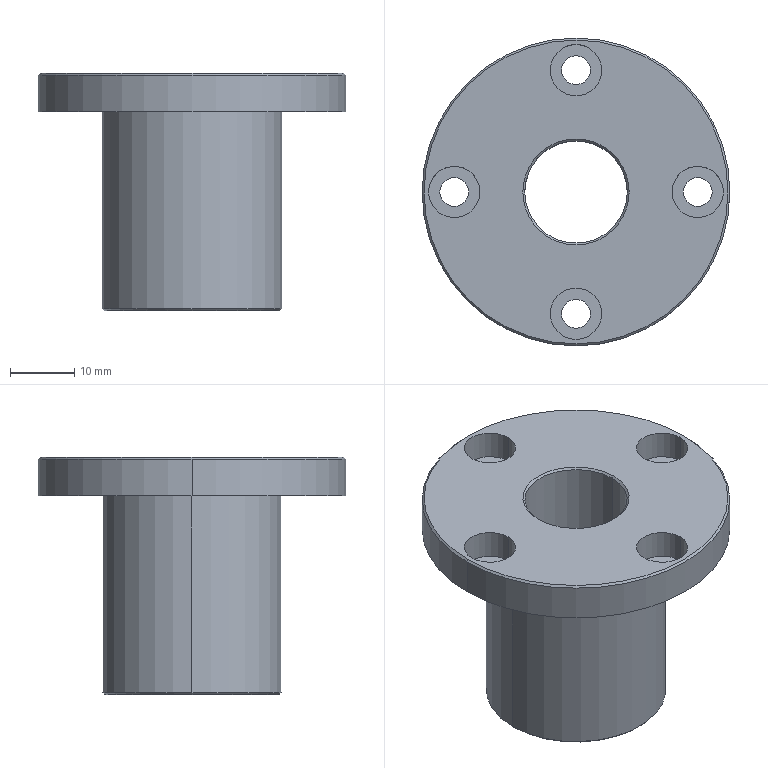Component | SolidWorks | LMF16UU(FlangedLinearBearing)-2 | 1 solid | 37 faces | box 48 x 48 x 37 mm | volume 21491 mm3 | cylinder 22 | cone 8 | plane 7 | commonest cylinder face diameters 8 x8 4.5 x8 16 x2 48 x2 28 x2
build123d program:
from build123d import *

# Parameters (mm, degrees)
SKETCH1_R                                            = 14
EXTRUDE1_DEPTH                                       = 18.5
SKETCH3_R                                            = 24
EXTRUDE3_DEPTH                                       = 6
SKETCH4_R                                            = 8
EXTRUDE4_DEPTH                                       = 51.21
HOLE_SIZE_ACCORDING_TO_TYPE_1_OF_HEXAGON_D           = 4.5
HOLE_SIZE_ACCORDING_TO_TYPE_1_OF_HEXAGON_CBORE_D     = 8
HOLE_SIZE_ACCORDING_TO_TYPE_1_OF_HEXAGON_CBORE_DEPTH = 4.5
CIRPATTERN1_COUNT                                    = 4
CHAMFER1_SIZE                                        = 0.3


with BuildPart() as part:
    # Sketch1 → Extrude1 (new, symmetric)
    with BuildSketch(Plane.XY):
        Circle(SKETCH1_R)
    extrude(amount=EXTRUDE1_DEPTH, both=True)

    # Sketch3 → Extrude3 (add)
    with BuildSketch(Plane(origin=(0, 0, -18.5), x_dir=(-1, 0, 0), z_dir=(0, 0, -1))):
        Circle(SKETCH3_R)
    extrude(amount=-EXTRUDE3_DEPTH)

    # Sketch4 → Extrude4 (cut, through all)
    with BuildSketch(Plane(origin=(0, 0, -18.5), x_dir=(-1, 0, 0), z_dir=(0, 0, -1))):
        Circle(SKETCH4_R)
    extrude(amount=-EXTRUDE4_DEPTH, mode=Mode.SUBTRACT)

    # Hole Size According to Type 1 of Hexagon (through all)
    with Locations(Plane(origin=(0, 0, -18.5), x_dir=(-1, 0, 0), z_dir=(0, 0, -1))):
        with Locations((0, 19)):
            hole_size_according_to_type_1_of_hexagon = CounterBoreHole(HOLE_SIZE_ACCORDING_TO_TYPE_1_OF_HEXAGON_D / 2, HOLE_SIZE_ACCORDING_TO_TYPE_1_OF_HEXAGON_CBORE_D / 2, HOLE_SIZE_ACCORDING_TO_TYPE_1_OF_HEXAGON_CBORE_DEPTH)

    # CirPattern1: Hole Size According to Type 1 of Hexagon ×4 about axis
    cirpattern1_axis = Axis((0, 0, 0), (0, 0, 1))
    for i in range(1, CIRPATTERN1_COUNT):
        add(hole_size_according_to_type_1_of_hexagon.rotate(cirpattern1_axis, i * 360 / CIRPATTERN1_COUNT), mode=Mode.SUBTRACT)

    # Chamfer1
    chamfer1_edges = [part.edges().sort_by_distance(p)[0] for p in [
        (8, 0, 18.5),
        (8, 0, -18.5),
        (-14, 0, 18.5),
        (24, 0, -18.5),
    ]]
    chamfer(chamfer1_edges, length=CHAMFER1_SIZE)


solid = part.part

# Placed as in the assembly
solid = solid.moved(Location((359.365, 247.727, 2019.633), (180, 0, 0)))